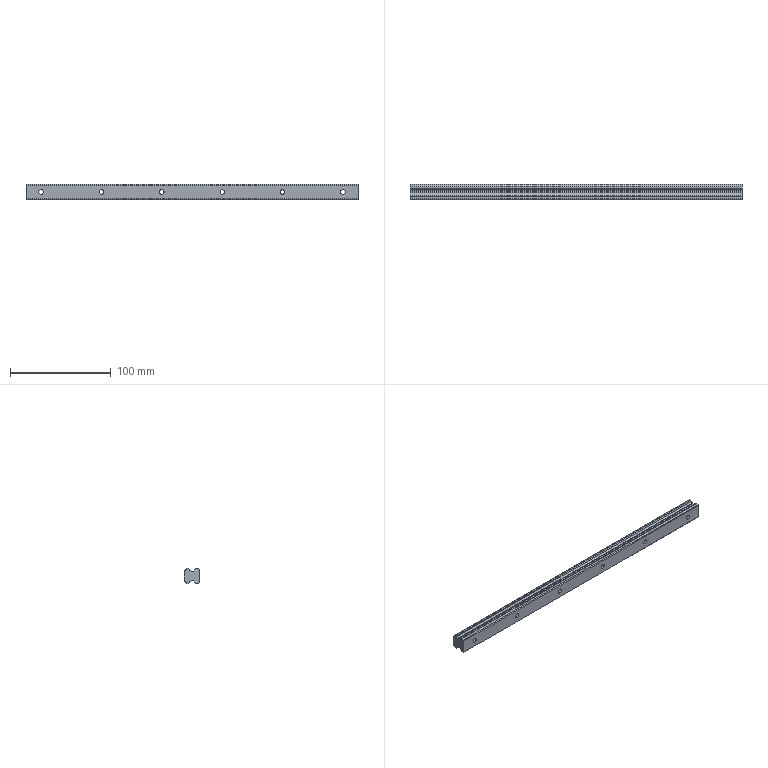Component | SolidWorks | HGH15CA-1_HGH_15_ASM_3_ASM-1_HGR15_1-1 | 1 solid | 66 faces | volume 60660 mm3 | cylinder 38 | plane 28 | commonest cylinder face diameters 0.8 x8 8 x6 4.3 x6 4.5 x6 7.5 x6 3.24 x4 2 x2